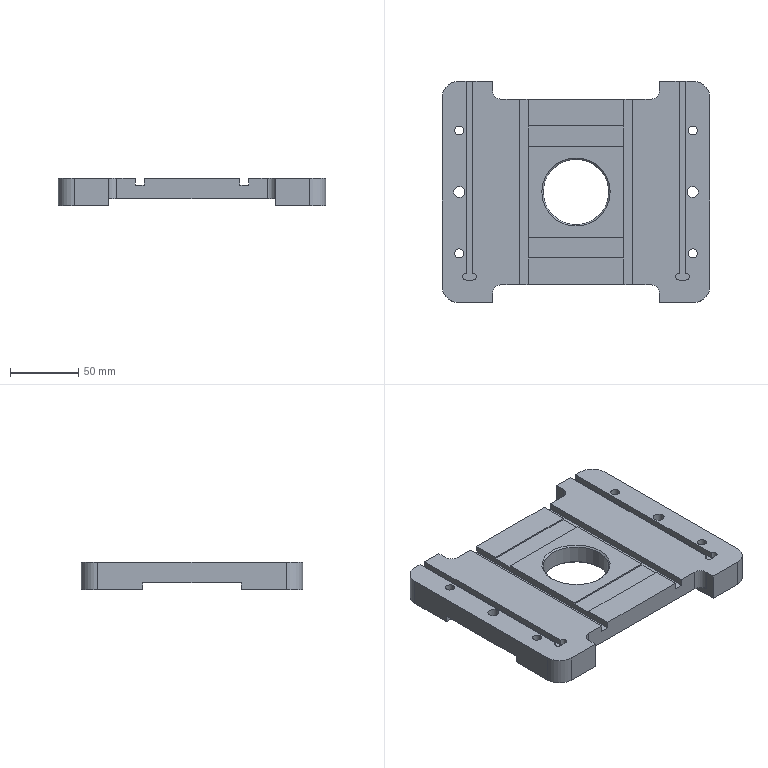Component | NX | BASE_PLATE | 1 solid | 97 faces | volume 384941 mm3 | plane 64 | cylinder 31 | cone 2 | commonest cylinder face diameters 12 x8 24 x4 5 x4 20 x4 6.6 x4 11 x4 8 x2 48 x1